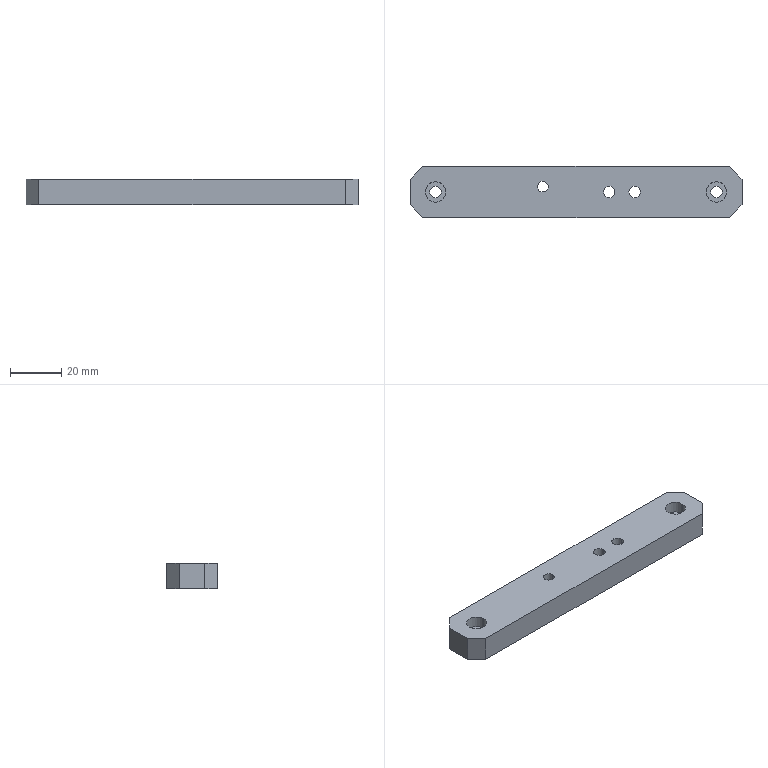Component | SolidWorks | P-SLJ-004-3_P-SLJ-004-003-1 | 1 solid | 32 faces | box 130 x 20 x 10 mm | volume 24093 mm3 | cylinder 18 | plane 14 | commonest cylinder face diameters 8 x8 4.5 x8 4.2 x2 | material A3
build123d program:
from build123d import *

# Parameters (mm, degrees)
SKETCH2_W                                            = 10
SKETCH2_H                                            = 20
EXTRUDE1_DEPTH                                       = 65
CBORE_FOR_M4_HEXAGON_SOCKET_HEAD_CAP_SCR_D           = 4.5
CBORE_FOR_M4_HEXAGON_SOCKET_HEAD_CAP_SCR_CBORE_D     = 8
CBORE_FOR_M4_HEXAGON_SOCKET_HEAD_CAP_SCR_CBORE_DEPTH = 4.6
M5_TAPPED_HOLE1_D                                    = 4.2
CBORE_FOR_M4_HEXAGON_SOCKET_HEAD_CAP_2_D             = 4.5
CBORE_FOR_M4_HEXAGON_SOCKET_HEAD_CAP_2_CBORE_D       = 8
CBORE_FOR_M4_HEXAGON_SOCKET_HEAD_CAP_2_CBORE_DEPTH   = 4.6
CHAMFER1_SIZE                                        = 5


with BuildPart() as part:
    # Sketch2 → Extrude1 (new, symmetric)
    with BuildSketch(Plane.XY):
        Rectangle(SKETCH2_W, SKETCH2_H)
    extrude(amount=EXTRUDE1_DEPTH, both=True)

    # CBORE for M4 Hexagon socket head cap scr (through all)
    with Locations(Plane.ZY.offset(5)):
        with Locations((-23, 0), (-13, 0)):
            CounterBoreHole(CBORE_FOR_M4_HEXAGON_SOCKET_HEAD_CAP_SCR_D / 2, CBORE_FOR_M4_HEXAGON_SOCKET_HEAD_CAP_SCR_CBORE_D / 2, CBORE_FOR_M4_HEXAGON_SOCKET_HEAD_CAP_SCR_CBORE_DEPTH)

    # M5 Tapped Hole1 (through all)
    with Locations(Plane.ZY.offset(5)):
        with Locations((13, 2.1)):
            Hole(M5_TAPPED_HOLE1_D / 2)

    # CBORE for M4 Hexagon socket head cap 2 (through all)
    with Locations(Plane(origin=(5, 2.408, 5.827), x_dir=(0, 0, 1), z_dir=(1, 0, 0))):
        with Locations((-60.827, 2.408), (49.173, 2.408)):
            CounterBoreHole(CBORE_FOR_M4_HEXAGON_SOCKET_HEAD_CAP_2_D / 2, CBORE_FOR_M4_HEXAGON_SOCKET_HEAD_CAP_2_CBORE_D / 2, CBORE_FOR_M4_HEXAGON_SOCKET_HEAD_CAP_2_CBORE_DEPTH)

    # Chamfer1
    chamfer1_edges = [part.edges().sort_by_distance(p)[0] for p in [
        (0, -10, 65),
        (0, -10, -65),
        (0, 10, -65),
        (0, 10, 65),
    ]]
    chamfer(chamfer1_edges, length=CHAMFER1_SIZE)


solid = part.part

# Placed as in the assembly
solid = solid.moved(Location((-219.5, -45, 1259.634), (0, -90, 0)))
STEP:
#1=CARTESIAN_POINT('',(-6.634,-1.772,49.608));
#2=VERTEX_POINT('',#1);
#3=CARTESIAN_POINT('',(-6.319,-1.772,49.608));
#4=VERTEX_POINT('',#3);
#5=CARTESIAN_POINT('',(-6.476,-1.772,49.608));
#6=DIRECTION('',(0.,-0.,1.));
#7=DIRECTION('',(1.,0.,0.));
#8=AXIS2_PLACEMENT_3D('',#5,#6,#7);
#9=CIRCLE('',#8,0.1575);
#10=EDGE_CURVE('',#2,#4,#9,.T.);
#11=ORIENTED_EDGE('',*,*,#10,.F.);
#12=CARTESIAN_POINT('',(-6.634,-1.772,49.789));
#13=VERTEX_POINT('',#12);
#14=CARTESIAN_POINT('',(-6.634,-1.772,49.789));
#15=DIRECTION('',(0.,-0.,1.));
#16=VECTOR('',#15,39.37);
#17=LINE('',#14,#16);
#18=EDGE_CURVE('',#2,#13,#17,.T.);
#19=ORIENTED_EDGE('',*,*,#18,.T.);
#20=CARTESIAN_POINT('',(-6.319,-1.772,49.789));
#21=VERTEX_POINT('',#20);
#22=CARTESIAN_POINT('',(-6.476,-1.772,49.789));
#23=DIRECTION('',(0.,-0.,1.));
#24=DIRECTION('',(1.,0.,0.));
#25=AXIS2_PLACEMENT_3D('',#22,#23,#24);
#26=CIRCLE('',#25,0.1575);
#27=EDGE_CURVE('',#13,#21,#26,.T.);
#28=ORIENTED_EDGE('',*,*,#27,.T.);
#29=CARTESIAN_POINT('',(-6.319,-1.772,49.789));
#30=DIRECTION('',(0.,-0.,1.));
#31=VECTOR('',#30,39.37);
#32=LINE('',#29,#31);
#33=EDGE_CURVE('',#4,#21,#32,.T.);
#34=ORIENTED_EDGE('',*,*,#33,.F.);
#35=EDGE_LOOP('',(#11,#19,#28,#34));
#36=FACE_OUTER_BOUND('',#35,.T.);
#37=CARTESIAN_POINT('',(-6.476,-1.772,49.789));
#38=DIRECTION('',(0.,-0.,1.));
#39=DIRECTION('',(1.,0.,0.));
#40=AXIS2_PLACEMENT_3D('',#37,#38,#39);
#41=CYLINDRICAL_SURFACE('',#40,0.1575);
#42=ADVANCED_FACE('',(#36),#41,.F.);
#43=CARTESIAN_POINT('',(-6.565,-1.772,49.395));
#44=VERTEX_POINT('',#43);
#45=CARTESIAN_POINT('',(-6.388,-1.772,49.395));
#46=VERTEX_POINT('',#45);
#47=CARTESIAN_POINT('',(-6.476,-1.772,49.395));
#48=DIRECTION('',(0.,-0.,1.));
#49=DIRECTION('',(1.,0.,0.));
#50=AXIS2_PLACEMENT_3D('',#47,#48,#49);
#51=CIRCLE('',#50,0.08858);
#52=EDGE_CURVE('',#44,#46,#51,.T.);
#53=ORIENTED_EDGE('',*,*,#52,.F.);
#54=CARTESIAN_POINT('',(-6.565,-1.772,49.608));
#55=VERTEX_POINT('',#54);
#56=CARTESIAN_POINT('',(-6.565,-1.772,49.789));
#57=DIRECTION('',(0.,-0.,1.));
#58=VECTOR('',#57,39.37);
#59=LINE('',#56,#58);
#60=EDGE_CURVE('',#44,#55,#59,.T.);
#61=ORIENTED_EDGE('',*,*,#60,.T.);
#62=CARTESIAN_POINT('',(-6.388,-1.772,49.608));
#63=VERTEX_POINT('',#62);
#64=CARTESIAN_POINT('',(-6.476,-1.772,49.608));
#65=DIRECTION('',(0.,-0.,1.));
#66=DIRECTION('',(1.,0.,0.));
#67=AXIS2_PLACEMENT_3D('',#64,#65,#66);
#68=CIRCLE('',#67,0.08858);
#69=EDGE_CURVE('',#55,#63,#68,.T.);
#70=ORIENTED_EDGE('',*,*,#69,.T.);
#71=CARTESIAN_POINT('',(-6.388,-1.772,49.789));
#72=DIRECTION('',(0.,-0.,1.));
#73=VECTOR('',#72,39.37);
#74=LINE('',#71,#73);
#75=EDGE_CURVE('',#46,#63,#74,.T.);
#76=ORIENTED_EDGE('',*,*,#75,.F.);
#77=EDGE_LOOP('',(#53,#61,#70,#76));
#78=FACE_OUTER_BOUND('',#77,.T.);
#79=CARTESIAN_POINT('',(-6.476,-1.772,49.789));
#80=DIRECTION('',(0.,-0.,1.));
#81=DIRECTION('',(1.,0.,0.));
#82=AXIS2_PLACEMENT_3D('',#79,#80,#81);
#83=CYLINDRICAL_SURFACE('',#82,0.08858);
#84=ADVANCED_FACE('',(#78),#83,.F.);
#85=CARTESIAN_POINT('',(-10.965,-1.772,49.608));
#86=VERTEX_POINT('',#85);
#87=CARTESIAN_POINT('',(-10.65,-1.772,49.608));
#88=VERTEX_POINT('',#87);
#89=CARTESIAN_POINT('',(-10.807,-1.772,49.608));
#90=DIRECTION('',(0.,-0.,1.));
#91=DIRECTION('',(1.,0.,0.));
#92=AXIS2_PLACEMENT_3D('',#89,#90,#91);
#93=CIRCLE('',#92,0.1575);
#94=EDGE_CURVE('',#86,#88,#93,.T.);
#95=ORIENTED_EDGE('',*,*,#94,.F.);
#96=CARTESIAN_POINT('',(-10.965,-1.772,49.789));
#97=VERTEX_POINT('',#96);
#98=CARTESIAN_POINT('',(-10.965,-1.772,49.789));
#99=DIRECTION('',(0.,-0.,1.));
#100=VECTOR('',#99,39.37);
#101=LINE('',#98,#100);
#102=EDGE_CURVE('',#86,#97,#101,.T.);
#103=ORIENTED_EDGE('',*,*,#102,.T.);
#104=CARTESIAN_POINT('',(-10.65,-1.772,49.789));
#105=VERTEX_POINT('',#104);
#106=CARTESIAN_POINT('',(-10.807,-1.772,49.789));
#107=DIRECTION('',(0.,-0.,1.));
#108=DIRECTION('',(1.,0.,0.));
#109=AXIS2_PLACEMENT_3D('',#106,#107,#108);
#110=CIRCLE('',#109,0.1575);
#111=EDGE_CURVE('',#97,#105,#110,.T.);
#112=ORIENTED_EDGE('',*,*,#111,.T.);
#113=CARTESIAN_POINT('',(-10.65,-1.772,49.789));
#114=DIRECTION('',(0.,-0.,1.));
#115=VECTOR('',#114,39.37);
#116=LINE('',#113,#115);
#117=EDGE_CURVE('',#88,#105,#116,.T.);
#118=ORIENTED_EDGE('',*,*,#117,.F.);
#119=EDGE_LOOP('',(#95,#103,#112,#118));
#120=FACE_OUTER_BOUND('',#119,.T.);
#121=CARTESIAN_POINT('',(-10.807,-1.772,49.789));
#122=DIRECTION('',(0.,-0.,1.));
#123=DIRECTION('',(1.,0.,0.));
#124=AXIS2_PLACEMENT_3D('',#121,#122,#123);
#125=CYLINDRICAL_SURFACE('',#124,0.1575);
#126=ADVANCED_FACE('',(#120),#125,.F.);
#127=CARTESIAN_POINT('',(-10.896,-1.772,49.395));
#128=VERTEX_POINT('',#127);
#129=CARTESIAN_POINT('',(-10.719,-1.772,49.395));
#130=VERTEX_POINT('',#129);
#131=CARTESIAN_POINT('',(-10.807,-1.772,49.395));
#132=DIRECTION('',(0.,-0.,1.));
#133=DIRECTION('',(1.,0.,0.));
#134=AXIS2_PLACEMENT_3D('',#131,#132,#133);
#135=CIRCLE('',#134,0.08858);
#136=EDGE_CURVE('',#128,#130,#135,.T.);
#137=ORIENTED_EDGE('',*,*,#136,.F.);
#138=CARTESIAN_POINT('',(-10.896,-1.772,49.608));
#139=VERTEX_POINT('',#138);
#140=CARTESIAN_POINT('',(-10.896,-1.772,49.789));
#141=DIRECTION('',(0.,-0.,1.));
#142=VECTOR('',#141,39.37);
#143=LINE('',#140,#142);
#144=EDGE_CURVE('',#128,#139,#143,.T.);
#145=ORIENTED_EDGE('',*,*,#144,.T.);
#146=CARTESIAN_POINT('',(-10.719,-1.772,49.608));
#147=VERTEX_POINT('',#146);
#148=CARTESIAN_POINT('',(-10.807,-1.772,49.608));
#149=DIRECTION('',(0.,-0.,1.));
#150=DIRECTION('',(1.,0.,0.));
#151=AXIS2_PLACEMENT_3D('',#148,#149,#150);
#152=CIRCLE('',#151,0.08858);
#153=EDGE_CURVE('',#139,#147,#152,.T.);
#154=ORIENTED_EDGE('',*,*,#153,.T.);
#155=CARTESIAN_POINT('',(-10.719,-1.772,49.789));
#156=DIRECTION('',(0.,-0.,1.));
#157=VECTOR('',#156,39.37);
#158=LINE('',#155,#157);
#159=EDGE_CURVE('',#130,#147,#158,.T.);
#160=ORIENTED_EDGE('',*,*,#159,.F.);
#161=EDGE_LOOP('',(#137,#145,#154,#160));
#162=FACE_OUTER_BOUND('',#161,.T.);
#163=CARTESIAN_POINT('',(-10.807,-1.772,49.789));
#164=DIRECTION('',(0.,-0.,1.));
#165=DIRECTION('',(1.,0.,0.));
#166=AXIS2_PLACEMENT_3D('',#163,#164,#165);
#167=CYLINDRICAL_SURFACE('',#166,0.08858);
#168=ADVANCED_FACE('',(#162),#167,.F.);
#169=CARTESIAN_POINT('',(-9.071,-1.689,49.789));
#170=VERTEX_POINT('',#169);
#171=CARTESIAN_POINT('',(-9.236,-1.689,49.789));
#172=VERTEX_POINT('',#171);
#173=CARTESIAN_POINT('',(-9.154,-1.689,49.789));
#174=DIRECTION('',(-0.,0.,-1.));
#175=DIRECTION('',(-1.,0.,0.));
#176=AXIS2_PLACEMENT_3D('',#173,#174,#175);
#177=CIRCLE('',#176,0.08268);
#178=EDGE_CURVE('',#170,#172,#177,.T.);
#179=ORIENTED_EDGE('',*,*,#178,.F.);
#180=CARTESIAN_POINT('',(-9.071,-1.689,49.395));
#181=VERTEX_POINT('',#180);
#182=CARTESIAN_POINT('',(-9.071,-1.689,49.395));
#183=DIRECTION('',(-0.,0.,-1.));
#184=VECTOR('',#183,39.37);
#185=LINE('',#182,#184);
#186=EDGE_CURVE('',#170,#181,#185,.T.);
#187=ORIENTED_EDGE('',*,*,#186,.T.);
#188=CARTESIAN_POINT('',(-9.236,-1.689,49.395));
#189=VERTEX_POINT('',#188);
#190=CARTESIAN_POINT('',(-9.154,-1.689,49.395));
#191=DIRECTION('',(-0.,0.,-1.));
#192=DIRECTION('',(-1.,0.,0.));
#193=AXIS2_PLACEMENT_3D('',#190,#191,#192);
#194=CIRCLE('',#193,0.08268);
#195=EDGE_CURVE('',#181,#189,#194,.T.);
#196=ORIENTED_EDGE('',*,*,#195,.T.);
#197=CARTESIAN_POINT('',(-9.236,-1.689,49.395));
#198=DIRECTION('',(-0.,0.,-1.));
#199=VECTOR('',#198,39.37);
#200=LINE('',#197,#199);
#201=EDGE_CURVE('',#172,#189,#200,.T.);
#202=ORIENTED_EDGE('',*,*,#201,.F.);
#203=EDGE_LOOP('',(#179,#187,#196,#202));
#204=FACE_OUTER_BOUND('',#203,.T.);
#205=CARTESIAN_POINT('',(-9.154,-1.689,49.395));
#206=DIRECTION('',(-0.,0.,-1.));
#207=DIRECTION('',(-1.,0.,0.));
#208=AXIS2_PLACEMENT_3D('',#205,#206,#207);
#209=CYLINDRICAL_SURFACE('',#208,0.08268);
#210=ADVANCED_FACE('',(#204),#209,.F.);
#211=CARTESIAN_POINT('',(-7.579,-1.772,49.576));
#212=VERTEX_POINT('',#211);
#213=CARTESIAN_POINT('',(-7.894,-1.772,49.576));
#214=VERTEX_POINT('',#213);
#215=CARTESIAN_POINT('',(-7.736,-1.772,49.576));
#216=DIRECTION('',(-0.,0.,-1.));
#217=DIRECTION('',(-1.,0.,0.));
#218=AXIS2_PLACEMENT_3D('',#215,#216,#217);
#219=CIRCLE('',#218,0.1575);
#220=EDGE_CURVE('',#212,#214,#219,.T.);
#221=ORIENTED_EDGE('',*,*,#220,.F.);
#222=CARTESIAN_POINT('',(-7.579,-1.772,49.395));
#223=VERTEX_POINT('',#222);
#224=CARTESIAN_POINT('',(-7.579,-1.772,49.395));
#225=DIRECTION('',(-0.,0.,-1.));
#226=VECTOR('',#225,39.37);
#227=LINE('',#224,#226);
#228=EDGE_CURVE('',#212,#223,#227,.T.);
#229=ORIENTED_EDGE('',*,*,#228,.T.);
#230=CARTESIAN_POINT('',(-7.894,-1.772,49.395));
#231=VERTEX_POINT('',#230);
#232=CARTESIAN_POINT('',(-7.736,-1.772,49.395));
#233=DIRECTION('',(-0.,0.,-1.));
#234=DIRECTION('',(-1.,0.,0.));
#235=AXIS2_PLACEMENT_3D('',#232,#233,#234);
#236=CIRCLE('',#235,0.1575);
#237=EDGE_CURVE('',#223,#231,#236,.T.);
#238=ORIENTED_EDGE('',*,*,#237,.T.);
#239=CARTESIAN_POINT('',(-7.894,-1.772,49.395));
#240=DIRECTION('',(-0.,0.,-1.));
#241=VECTOR('',#240,39.37);
#242=LINE('',#239,#241);
#243=EDGE_CURVE('',#214,#231,#242,.T.);
#244=ORIENTED_EDGE('',*,*,#243,.F.);
#245=EDGE_LOOP('',(#221,#229,#238,#244));
#246=FACE_OUTER_BOUND('',#245,.T.);
#247=CARTESIAN_POINT('',(-7.736,-1.772,49.395));
#248=DIRECTION('',(-0.,0.,-1.));
#249=DIRECTION('',(-1.,0.,0.));
#250=AXIS2_PLACEMENT_3D('',#247,#248,#249);
#251=CYLINDRICAL_SURFACE('',#250,0.1575);
#252=ADVANCED_FACE('',(#246),#251,.F.);
#253=CARTESIAN_POINT('',(-7.648,-1.772,49.789));
#254=VERTEX_POINT('',#253);
#255=CARTESIAN_POINT('',(-7.825,-1.772,49.789));
#256=VERTEX_POINT('',#255);
#257=CARTESIAN_POINT('',(-7.736,-1.772,49.789));
#258=DIRECTION('',(-0.,0.,-1.));
#259=DIRECTION('',(-1.,0.,0.));
#260=AXIS2_PLACEMENT_3D('',#257,#258,#259);
#261=CIRCLE('',#260,0.08858);
#262=EDGE_CURVE('',#254,#256,#261,.T.);
#263=ORIENTED_EDGE('',*,*,#262,.F.);
#264=CARTESIAN_POINT('',(-7.648,-1.772,49.576));
#265=VERTEX_POINT('',#264);
#266=CARTESIAN_POINT('',(-7.648,-1.772,49.395));
#267=DIRECTION('',(-0.,0.,-1.));
#268=VECTOR('',#267,39.37);
#269=LINE('',#266,#268);
#270=EDGE_CURVE('',#254,#265,#269,.T.);
#271=ORIENTED_EDGE('',*,*,#270,.T.);
#272=CARTESIAN_POINT('',(-7.825,-1.772,49.576));
#273=VERTEX_POINT('',#272);
#274=CARTESIAN_POINT('',(-7.736,-1.772,49.576));
#275=DIRECTION('',(-0.,0.,-1.));
#276=DIRECTION('',(-1.,0.,0.));
#277=AXIS2_PLACEMENT_3D('',#274,#275,#276);
#278=CIRCLE('',#277,0.08858);
#279=EDGE_CURVE('',#265,#273,#278,.T.);
#280=ORIENTED_EDGE('',*,*,#279,.T.);
#281=CARTESIAN_POINT('',(-7.825,-1.772,49.395));
#282=DIRECTION('',(-0.,0.,-1.));
#283=VECTOR('',#282,39.37);
#284=LINE('',#281,#283);
#285=EDGE_CURVE('',#256,#273,#284,.T.);
#286=ORIENTED_EDGE('',*,*,#285,.F.);
#287=EDGE_LOOP('',(#263,#271,#280,#286));
#288=FACE_OUTER_BOUND('',#287,.T.);
#289=CARTESIAN_POINT('',(-7.736,-1.772,49.395));
#290=DIRECTION('',(-0.,0.,-1.));
#291=DIRECTION('',(-1.,0.,0.));
#292=AXIS2_PLACEMENT_3D('',#289,#290,#291);
#293=CYLINDRICAL_SURFACE('',#292,0.08858);
#294=ADVANCED_FACE('',(#288),#293,.F.);
#295=CARTESIAN_POINT('',(-7.972,-1.772,49.576));
#296=VERTEX_POINT('',#295);
#297=CARTESIAN_POINT('',(-8.287,-1.772,49.576));
#298=VERTEX_POINT('',#297);
#299=CARTESIAN_POINT('',(-8.13,-1.772,49.576));
#300=DIRECTION('',(-0.,0.,-1.));
#301=DIRECTION('',(-1.,0.,0.));
#302=AXIS2_PLACEMENT_3D('',#299,#300,#301);
#303=CIRCLE('',#302,0.1575);
#304=EDGE_CURVE('',#296,#298,#303,.T.);
#305=ORIENTED_EDGE('',*,*,#304,.F.);
#306=CARTESIAN_POINT('',(-7.972,-1.772,49.395));
#307=VERTEX_POINT('',#306);
#308=CARTESIAN_POINT('',(-7.972,-1.772,49.395));
#309=DIRECTION('',(-0.,0.,-1.));
#310=VECTOR('',#309,39.37);
#311=LINE('',#308,#310);
#312=EDGE_CURVE('',#296,#307,#311,.T.);
#313=ORIENTED_EDGE('',*,*,#312,.T.);
#314=CARTESIAN_POINT('',(-8.287,-1.772,49.395));
#315=VERTEX_POINT('',#314);
#316=CARTESIAN_POINT('',(-8.13,-1.772,49.395));
#317=DIRECTION('',(-0.,0.,-1.));
#318=DIRECTION('',(-1.,0.,0.));
#319=AXIS2_PLACEMENT_3D('',#316,#317,#318);
#320=CIRCLE('',#319,0.1575);
#321=EDGE_CURVE('',#307,#315,#320,.T.);
#322=ORIENTED_EDGE('',*,*,#321,.T.);
#323=CARTESIAN_POINT('',(-8.287,-1.772,49.395));
#324=DIRECTION('',(-0.,0.,-1.));
#325=VECTOR('',#324,39.37);
#326=LINE('',#323,#325);
#327=EDGE_CURVE('',#298,#315,#326,.T.);
#328=ORIENTED_EDGE('',*,*,#327,.F.);
#329=EDGE_LOOP('',(#305,#313,#322,#328));
#330=FACE_OUTER_BOUND('',#329,.T.);
#331=CARTESIAN_POINT('',(-8.13,-1.772,49.395));
#332=DIRECTION('',(-0.,0.,-1.));
#333=DIRECTION('',(-1.,0.,0.));
#334=AXIS2_PLACEMENT_3D('',#331,#332,#333);
#335=CYLINDRICAL_SURFACE('',#334,0.1575);
#336=ADVANCED_FACE('',(#330),#335,.F.);
#337=CARTESIAN_POINT('',(-8.041,-1.772,49.789));
#338=VERTEX_POINT('',#337);
#339=CARTESIAN_POINT('',(-8.219,-1.772,49.789));
#340=VERTEX_POINT('',#339);
#341=CARTESIAN_POINT('',(-8.13,-1.772,49.789));
#342=DIRECTION('',(-0.,0.,-1.));
#343=DIRECTION('',(-1.,0.,0.));
#344=AXIS2_PLACEMENT_3D('',#341,#342,#343);
#345=CIRCLE('',#344,0.08858);
#346=EDGE_CURVE('',#338,#340,#345,.T.);
#347=ORIENTED_EDGE('',*,*,#346,.F.);
#348=CARTESIAN_POINT('',(-8.041,-1.772,49.576));
#349=VERTEX_POINT('',#348);
#350=CARTESIAN_POINT('',(-8.041,-1.772,49.395));
#351=DIRECTION('',(-0.,0.,-1.));
#352=VECTOR('',#351,39.37);
#353=LINE('',#350,#352);
#354=EDGE_CURVE('',#338,#349,#353,.T.);
#355=ORIENTED_EDGE('',*,*,#354,.T.);
#356=CARTESIAN_POINT('',(-8.219,-1.772,49.576));
#357=VERTEX_POINT('',#356);
#358=CARTESIAN_POINT('',(-8.13,-1.772,49.576));
#359=DIRECTION('',(-0.,0.,-1.));
#360=DIRECTION('',(-1.,0.,0.));
#361=AXIS2_PLACEMENT_3D('',#358,#359,#360);
#362=CIRCLE('',#361,0.08858);
#363=EDGE_CURVE('',#349,#357,#362,.T.);
#364=ORIENTED_EDGE('',*,*,#363,.T.);
#365=CARTESIAN_POINT('',(-8.219,-1.772,49.395));
#366=DIRECTION('',(-0.,0.,-1.));
#367=VECTOR('',#366,39.37);
#368=LINE('',#365,#367);
#369=EDGE_CURVE('',#340,#357,#368,.T.);
#370=ORIENTED_EDGE('',*,*,#369,.F.);
#371=EDGE_LOOP('',(#347,#355,#364,#370));
#372=FACE_OUTER_BOUND('',#371,.T.);
#373=CARTESIAN_POINT('',(-8.13,-1.772,49.395));
#374=DIRECTION('',(-0.,0.,-1.));
#375=DIRECTION('',(-1.,0.,0.));
#376=AXIS2_PLACEMENT_3D('',#373,#374,#375);
#377=CYLINDRICAL_SURFACE('',#376,0.08858);
#378=ADVANCED_FACE('',(#372),#377,.F.);
#379=CARTESIAN_POINT('',(-6.476,-1.772,49.789));
#380=DIRECTION('',(0.,-0.,1.));
#381=DIRECTION('',(1.,0.,0.));
#382=AXIS2_PLACEMENT_3D('',#379,#380,#381);
#383=CIRCLE('',#382,0.1575);
#384=EDGE_CURVE('',#21,#13,#383,.T.);
#385=ORIENTED_EDGE('',*,*,#384,.F.);
#386=ORIENTED_EDGE('',*,*,#27,.F.);
#387=EDGE_LOOP('',(#385,#386));
#388=FACE_BOUND('',#387,.T.);
#389=CARTESIAN_POINT('',(-10.807,-1.772,49.789));
#390=DIRECTION('',(0.,-0.,1.));
#391=DIRECTION('',(1.,0.,0.));
#392=AXIS2_PLACEMENT_3D('',#389,#390,#391);
#393=CIRCLE('',#392,0.1575);
#394=EDGE_CURVE('',#105,#97,#393,.T.);
#395=ORIENTED_EDGE('',*,*,#394,.F.);
#396=ORIENTED_EDGE('',*,*,#111,.F.);
#397=EDGE_LOOP('',(#395,#396));
#398=FACE_BOUND('',#397,.T.);
#399=CARTESIAN_POINT('',(-9.154,-1.689,49.789));
#400=DIRECTION('',(-0.,0.,-1.));
#401=DIRECTION('',(-1.,0.,0.));
#402=AXIS2_PLACEMENT_3D('',#399,#400,#401);
#403=CIRCLE('',#402,0.08268);
#404=EDGE_CURVE('',#172,#170,#403,.T.);
#405=ORIENTED_EDGE('',*,*,#404,.T.);
#406=ORIENTED_EDGE('',*,*,#178,.T.);
#407=EDGE_LOOP('',(#405,#406));
#408=FACE_BOUND('',#407,.T.);
#409=CARTESIAN_POINT('',(-7.736,-1.772,49.789));
#410=DIRECTION('',(-0.,0.,-1.));
#411=DIRECTION('',(-1.,0.,0.));
#412=AXIS2_PLACEMENT_3D('',#409,#410,#411);
#413=CIRCLE('',#412,0.08858);
#414=EDGE_CURVE('',#256,#254,#413,.T.);
#415=ORIENTED_EDGE('',*,*,#414,.T.);
#416=ORIENTED_EDGE('',*,*,#262,.T.);
#417=EDGE_LOOP('',(#415,#416));
#418=FACE_BOUND('',#417,.T.);
#419=CARTESIAN_POINT('',(-8.13,-1.772,49.789));
#420=DIRECTION('',(-0.,0.,-1.));
#421=DIRECTION('',(-1.,0.,0.));
#422=AXIS2_PLACEMENT_3D('',#419,#420,#421);
#423=CIRCLE('',#422,0.08858);
#424=EDGE_CURVE('',#340,#338,#423,.T.);
#425=ORIENTED_EDGE('',*,*,#424,.T.);
#426=ORIENTED_EDGE('',*,*,#346,.T.);
#427=EDGE_LOOP('',(#425,#426));
#428=FACE_BOUND('',#427,.T.);
#429=CARTESIAN_POINT('',(-11.201,-1.969,49.789));
#430=VERTEX_POINT('',#429);
#431=CARTESIAN_POINT('',(-11.201,-1.575,49.789));
#432=VERTEX_POINT('',#431);
#433=CARTESIAN_POINT('',(-11.201,-2.165,49.789));
#434=DIRECTION('',(0.,1.,0.));
#435=VECTOR('',#434,39.37);
#436=LINE('',#433,#435);
#437=EDGE_CURVE('',#430,#432,#436,.T.);
#438=ORIENTED_EDGE('',*,*,#437,.F.);
#439=CARTESIAN_POINT('',(-11.004,-2.165,49.789));
#440=VERTEX_POINT('',#439);
#441=CARTESIAN_POINT('',(-11.201,-1.969,49.789));
#442=DIRECTION('',(0.7071,-0.7071,-0.));
#443=VECTOR('',#442,39.37);
#444=LINE('',#441,#443);
#445=EDGE_CURVE('',#430,#440,#444,.T.);
#446=ORIENTED_EDGE('',*,*,#445,.T.);
#447=CARTESIAN_POINT('',(-6.28,-2.165,49.789));
#448=VERTEX_POINT('',#447);
#449=CARTESIAN_POINT('',(-11.201,-2.165,49.789));
#450=DIRECTION('',(1.,-0.,-0.));
#451=VECTOR('',#450,39.37);
#452=LINE('',#449,#451);
#453=EDGE_CURVE('',#440,#448,#452,.T.);
#454=ORIENTED_EDGE('',*,*,#453,.T.);
#455=CARTESIAN_POINT('',(-6.083,-1.969,49.789));
#456=VERTEX_POINT('',#455);
#457=CARTESIAN_POINT('',(-6.28,-2.165,49.789));
#458=DIRECTION('',(0.7071,0.7071,0.));
#459=VECTOR('',#458,39.37);
#460=LINE('',#457,#459);
#461=EDGE_CURVE('',#448,#456,#460,.T.);
#462=ORIENTED_EDGE('',*,*,#461,.T.);
#463=CARTESIAN_POINT('',(-6.083,-1.575,49.789));
#464=VERTEX_POINT('',#463);
#465=CARTESIAN_POINT('',(-6.083,-2.165,49.789));
#466=DIRECTION('',(0.,1.,0.));
#467=VECTOR('',#466,39.37);
#468=LINE('',#465,#467);
#469=EDGE_CURVE('',#456,#464,#468,.T.);
#470=ORIENTED_EDGE('',*,*,#469,.T.);
#471=CARTESIAN_POINT('',(-6.28,-1.378,49.789));
#472=VERTEX_POINT('',#471);
#473=CARTESIAN_POINT('',(-6.28,-1.378,49.789));
#474=DIRECTION('',(-0.7071,0.7071,0.));
#475=VECTOR('',#474,39.37);
#476=LINE('',#473,#475);
#477=EDGE_CURVE('',#464,#472,#476,.T.);
#478=ORIENTED_EDGE('',*,*,#477,.T.);
#479=CARTESIAN_POINT('',(-11.004,-1.378,49.789));
#480=VERTEX_POINT('',#479);
#481=CARTESIAN_POINT('',(-11.201,-1.378,49.789));
#482=DIRECTION('',(1.,-0.,-0.));
#483=VECTOR('',#482,39.37);
#484=LINE('',#481,#483);
#485=EDGE_CURVE('',#480,#472,#484,.T.);
#486=ORIENTED_EDGE('',*,*,#485,.F.);
#487=CARTESIAN_POINT('',(-11.201,-1.575,49.789));
#488=DIRECTION('',(-0.7071,-0.7071,-0.));
#489=VECTOR('',#488,39.37);
#490=LINE('',#487,#489);
#491=EDGE_CURVE('',#480,#432,#490,.T.);
#492=ORIENTED_EDGE('',*,*,#491,.T.);
#493=EDGE_LOOP('',(#438,#446,#454,#462,#470,#478,#486,#492));
#494=FACE_OUTER_BOUND('',#493,.T.);
#495=CARTESIAN_POINT('',(-11.201,-2.165,49.789));
#496=DIRECTION('',(-0.,0.,-1.));
#497=DIRECTION('',(-1.,0.,0.));
#498=AXIS2_PLACEMENT_3D('',#495,#496,#497);
#499=PLANE('',#498);
#500=ADVANCED_FACE('',(#388,#398,#408,#418,#428,#494),#499,.F.);
#501=CARTESIAN_POINT('',(-11.004,-1.378,49.395));
#502=VERTEX_POINT('',#501);
#503=CARTESIAN_POINT('',(-6.28,-1.378,49.395));
#504=VERTEX_POINT('',#503);
#505=CARTESIAN_POINT('',(-11.201,-1.378,49.395));
#506=DIRECTION('',(1.,-0.,-0.));
#507=VECTOR('',#506,39.37);
#508=LINE('',#505,#507);
#509=EDGE_CURVE('',#502,#504,#508,.T.);
#510=ORIENTED_EDGE('',*,*,#509,.F.);
#511=CARTESIAN_POINT('',(-11.004,-1.378,49.395));
#512=DIRECTION('',(0.,-0.,1.));
#513=VECTOR('',#512,39.37);
#514=LINE('',#511,#513);
#515=EDGE_CURVE('',#502,#480,#514,.T.);
#516=ORIENTED_EDGE('',*,*,#515,.T.);
#517=ORIENTED_EDGE('',*,*,#485,.T.);
#518=CARTESIAN_POINT('',(-6.28,-1.378,49.395));
#519=DIRECTION('',(-0.,0.,-1.));
#520=VECTOR('',#519,39.37);
#521=LINE('',#518,#520);
#522=EDGE_CURVE('',#472,#504,#521,.T.);
#523=ORIENTED_EDGE('',*,*,#522,.T.);
#524=EDGE_LOOP('',(#510,#516,#517,#523));
#525=FACE_OUTER_BOUND('',#524,.T.);
#526=CARTESIAN_POINT('',(-11.201,-1.378,49.395));
#527=DIRECTION('',(-0.,-1.,-0.));
#528=DIRECTION('',(1.,-0.,-0.));
#529=AXIS2_PLACEMENT_3D('',#526,#527,#528);
#530=PLANE('',#529);
#531=ADVANCED_FACE('',(#525),#530,.F.);
#532=CARTESIAN_POINT('',(-6.476,-1.772,49.395));
#533=DIRECTION('',(0.,-0.,1.));
#534=DIRECTION('',(1.,0.,0.));
#535=AXIS2_PLACEMENT_3D('',#532,#533,#534);
#536=CIRCLE('',#535,0.08858);
#537=EDGE_CURVE('',#46,#44,#536,.T.);
#538=ORIENTED_EDGE('',*,*,#537,.T.);
#539=ORIENTED_EDGE('',*,*,#52,.T.);
#540=EDGE_LOOP('',(#538,#539));
#541=FACE_BOUND('',#540,.T.);
#542=CARTESIAN_POINT('',(-10.807,-1.772,49.395));
#543=DIRECTION('',(0.,-0.,1.));
#544=DIRECTION('',(1.,0.,0.));
#545=AXIS2_PLACEMENT_3D('',#542,#543,#544);
#546=CIRCLE('',#545,0.08858);
#547=EDGE_CURVE('',#130,#128,#546,.T.);
#548=ORIENTED_EDGE('',*,*,#547,.T.);
#549=ORIENTED_EDGE('',*,*,#136,.T.);
#550=EDGE_LOOP('',(#548,#549));
#551=FACE_BOUND('',#550,.T.);
#552=CARTESIAN_POINT('',(-9.154,-1.689,49.395));
#553=DIRECTION('',(-0.,0.,-1.));
#554=DIRECTION('',(-1.,0.,0.));
#555=AXIS2_PLACEMENT_3D('',#552,#553,#554);
#556=CIRCLE('',#555,0.08268);
#557=EDGE_CURVE('',#189,#181,#556,.T.);
#558=ORIENTED_EDGE('',*,*,#557,.F.);
#559=ORIENTED_EDGE('',*,*,#195,.F.);
#560=EDGE_LOOP('',(#558,#559));
#561=FACE_BOUND('',#560,.T.);
#562=CARTESIAN_POINT('',(-7.736,-1.772,49.395));
#563=DIRECTION('',(-0.,0.,-1.));
#564=DIRECTION('',(-1.,0.,0.));
#565=AXIS2_PLACEMENT_3D('',#562,#563,#564);
#566=CIRCLE('',#565,0.1575);
#567=EDGE_CURVE('',#231,#223,#566,.T.);
#568=ORIENTED_EDGE('',*,*,#567,.F.);
#569=ORIENTED_EDGE('',*,*,#237,.F.);
#570=EDGE_LOOP('',(#568,#569));
#571=FACE_BOUND('',#570,.T.);
#572=CARTESIAN_POINT('',(-8.13,-1.772,49.395));
#573=DIRECTION('',(-0.,0.,-1.));
#574=DIRECTION('',(-1.,0.,0.));
#575=AXIS2_PLACEMENT_3D('',#572,#573,#574);
#576=CIRCLE('',#575,0.1575);
#577=EDGE_CURVE('',#315,#307,#576,.T.);
#578=ORIENTED_EDGE('',*,*,#577,.F.);
#579=ORIENTED_EDGE('',*,*,#321,.F.);
#580=EDGE_LOOP('',(#578,#579));
#581=FACE_BOUND('',#580,.T.);
#582=CARTESIAN_POINT('',(-11.004,-2.165,49.395));
#583=VERTEX_POINT('',#582);
#584=CARTESIAN_POINT('',(-6.28,-2.165,49.395));
#585=VERTEX_POINT('',#584);
#586=CARTESIAN_POINT('',(-11.201,-2.165,49.395));
#587=DIRECTION('',(1.,-0.,-0.));
#588=VECTOR('',#587,39.37);
#589=LINE('',#586,#588);
#590=EDGE_CURVE('',#583,#585,#589,.T.);
#591=ORIENTED_EDGE('',*,*,#590,.F.);
#592=CARTESIAN_POINT('',(-11.201,-1.969,49.395));
#593=VERTEX_POINT('',#592);
#594=CARTESIAN_POINT('',(-11.201,-1.969,49.395));
#595=DIRECTION('',(-0.7071,0.7071,0.));
#596=VECTOR('',#595,39.37);
#597=LINE('',#594,#596);
#598=EDGE_CURVE('',#583,#593,#597,.T.);
#599=ORIENTED_EDGE('',*,*,#598,.T.);
#600=CARTESIAN_POINT('',(-11.201,-1.575,49.395));
#601=VERTEX_POINT('',#600);
#602=CARTESIAN_POINT('',(-11.201,-2.165,49.395));
#603=DIRECTION('',(-0.,-1.,-0.));
#604=VECTOR('',#603,39.37);
#605=LINE('',#602,#604);
#606=EDGE_CURVE('',#601,#593,#605,.T.);
#607=ORIENTED_EDGE('',*,*,#606,.F.);
#608=CARTESIAN_POINT('',(-11.201,-1.575,49.395));
#609=DIRECTION('',(0.7071,0.7071,0.));
#610=VECTOR('',#609,39.37);
#611=LINE('',#608,#610);
#612=EDGE_CURVE('',#601,#502,#611,.T.);
#613=ORIENTED_EDGE('',*,*,#612,.T.);
#614=ORIENTED_EDGE('',*,*,#509,.T.);
#615=CARTESIAN_POINT('',(-6.083,-1.575,49.395));
#616=VERTEX_POINT('',#615);
#617=CARTESIAN_POINT('',(-6.28,-1.378,49.395));
#618=DIRECTION('',(0.7071,-0.7071,-0.));
#619=VECTOR('',#618,39.37);
#620=LINE('',#617,#619);
#621=EDGE_CURVE('',#504,#616,#620,.T.);
#622=ORIENTED_EDGE('',*,*,#621,.T.);
#623=CARTESIAN_POINT('',(-6.083,-1.969,49.395));
#624=VERTEX_POINT('',#623);
#625=CARTESIAN_POINT('',(-6.083,-2.165,49.395));
#626=DIRECTION('',(-0.,-1.,-0.));
#627=VECTOR('',#626,39.37);
#628=LINE('',#625,#627);
#629=EDGE_CURVE('',#616,#624,#628,.T.);
#630=ORIENTED_EDGE('',*,*,#629,.T.);
#631=CARTESIAN_POINT('',(-6.28,-2.165,49.395));
#632=DIRECTION('',(-0.7071,-0.7071,-0.));
#633=VECTOR('',#632,39.37);
#634=LINE('',#631,#633);
#635=EDGE_CURVE('',#624,#585,#634,.T.);
#636=ORIENTED_EDGE('',*,*,#635,.T.);
#637=EDGE_LOOP('',(#591,#599,#607,#613,#614,#622,#630,#636));
#638=FACE_OUTER_BOUND('',#637,.T.);
#639=CARTESIAN_POINT('',(-11.201,-2.165,49.395));
#640=DIRECTION('',(0.,-0.,1.));
#641=DIRECTION('',(1.,-0.,-0.));
#642=AXIS2_PLACEMENT_3D('',#639,#640,#641);
#643=PLANE('',#642);
#644=ADVANCED_FACE('',(#541,#551,#561,#571,#581,#638),#643,.F.);
#645=ORIENTED_EDGE('',*,*,#453,.F.);
#646=CARTESIAN_POINT('',(-11.004,-2.165,49.395));
#647=DIRECTION('',(-0.,0.,-1.));
#648=VECTOR('',#647,39.37);
#649=LINE('',#646,#648);
#650=EDGE_CURVE('',#440,#583,#649,.T.);
#651=ORIENTED_EDGE('',*,*,#650,.T.);
#652=ORIENTED_EDGE('',*,*,#590,.T.);
#653=CARTESIAN_POINT('',(-6.28,-2.165,49.789));
#654=DIRECTION('',(0.,-0.,1.));
#655=VECTOR('',#654,39.37);
#656=LINE('',#653,#655);
#657=EDGE_CURVE('',#585,#448,#656,.T.);
#658=ORIENTED_EDGE('',*,*,#657,.T.);
#659=EDGE_LOOP('',(#645,#651,#652,#658));
#660=FACE_OUTER_BOUND('',#659,.T.);
#661=CARTESIAN_POINT('',(-11.201,-2.165,49.395));
#662=DIRECTION('',(0.,1.,0.));
#663=DIRECTION('',(-1.,0.,0.));
#664=AXIS2_PLACEMENT_3D('',#661,#662,#663);
#665=PLANE('',#664);
#666=ADVANCED_FACE('',(#660),#665,.F.);
#667=ORIENTED_EDGE('',*,*,#606,.T.);
#668=CARTESIAN_POINT('',(-11.201,-1.969,49.592));
#669=DIRECTION('',(0.,-0.,1.));
#670=VECTOR('',#669,39.37);
#671=LINE('',#668,#670);
#672=EDGE_CURVE('',#593,#430,#671,.T.);
#673=ORIENTED_EDGE('',*,*,#672,.T.);
#674=ORIENTED_EDGE('',*,*,#437,.T.);
#675=CARTESIAN_POINT('',(-11.201,-1.575,49.592));
#676=DIRECTION('',(-0.,0.,-1.));
#677=VECTOR('',#676,39.37);
#678=LINE('',#675,#677);
#679=EDGE_CURVE('',#432,#601,#678,.T.);
#680=ORIENTED_EDGE('',*,*,#679,.T.);
#681=EDGE_LOOP('',(#667,#673,#674,#680));
#682=FACE_OUTER_BOUND('',#681,.T.);
#683=CARTESIAN_POINT('',(-11.201,-1.772,49.592));
#684=DIRECTION('',(1.,-0.,-0.));
#685=DIRECTION('',(-0.,0.,-1.));
#686=AXIS2_PLACEMENT_3D('',#683,#684,#685);
#687=PLANE('',#686);
#688=ADVANCED_FACE('',(#682),#687,.F.);
#689=ORIENTED_EDGE('',*,*,#469,.F.);
#690=CARTESIAN_POINT('',(-6.083,-1.969,49.395));
#691=DIRECTION('',(-0.,0.,-1.));
#692=VECTOR('',#691,39.37);
#693=LINE('',#690,#692);
#694=EDGE_CURVE('',#456,#624,#693,.T.);
#695=ORIENTED_EDGE('',*,*,#694,.T.);
#696=ORIENTED_EDGE('',*,*,#629,.F.);
#697=CARTESIAN_POINT('',(-6.083,-1.575,49.789));
#698=DIRECTION('',(0.,-0.,1.));
#699=VECTOR('',#698,39.37);
#700=LINE('',#697,#699);
#701=EDGE_CURVE('',#616,#464,#700,.T.);
#702=ORIENTED_EDGE('',*,*,#701,.T.);
#703=EDGE_LOOP('',(#689,#695,#696,#702));
#704=FACE_OUTER_BOUND('',#703,.T.);
#705=CARTESIAN_POINT('',(-6.083,-1.772,49.592));
#706=DIRECTION('',(1.,-0.,-0.));
#707=DIRECTION('',(-0.,0.,-1.));
#708=AXIS2_PLACEMENT_3D('',#705,#706,#707);
#709=PLANE('',#708);
#710=ADVANCED_FACE('',(#704),#709,.T.);
#711=ORIENTED_EDGE('',*,*,#354,.F.);
#712=ORIENTED_EDGE('',*,*,#424,.F.);
#713=ORIENTED_EDGE('',*,*,#369,.T.);
#714=CARTESIAN_POINT('',(-8.13,-1.772,49.576));
#715=DIRECTION('',(-0.,0.,-1.));
#716=DIRECTION('',(-1.,0.,0.));
#717=AXIS2_PLACEMENT_3D('',#714,#715,#716);
#718=CIRCLE('',#717,0.08858);
#719=EDGE_CURVE('',#357,#349,#718,.T.);
#720=ORIENTED_EDGE('',*,*,#719,.T.);
#721=EDGE_LOOP('',(#711,#712,#713,#720));
#722=FACE_OUTER_BOUND('',#721,.T.);
#723=CARTESIAN_POINT('',(-8.13,-1.772,49.395));
#724=DIRECTION('',(-0.,0.,-1.));
#725=DIRECTION('',(-1.,0.,0.));
#726=AXIS2_PLACEMENT_3D('',#723,#724,#725);
#727=CYLINDRICAL_SURFACE('',#726,0.08858);
#728=ADVANCED_FACE('',(#722),#727,.F.);
#729=ORIENTED_EDGE('',*,*,#719,.F.);
#730=ORIENTED_EDGE('',*,*,#363,.F.);
#731=EDGE_LOOP('',(#729,#730));
#732=FACE_BOUND('',#731,.T.);
#733=CARTESIAN_POINT('',(-8.13,-1.772,49.576));
#734=DIRECTION('',(-0.,0.,-1.));
#735=DIRECTION('',(-1.,0.,0.));
#736=AXIS2_PLACEMENT_3D('',#733,#734,#735);
#737=CIRCLE('',#736,0.1575);
#738=EDGE_CURVE('',#298,#296,#737,.T.);
#739=ORIENTED_EDGE('',*,*,#738,.T.);
#740=ORIENTED_EDGE('',*,*,#304,.T.);
#741=EDGE_LOOP('',(#739,#740));
#742=FACE_OUTER_BOUND('',#741,.T.);
#743=CARTESIAN_POINT('',(-8.13,-1.683,49.576));
#744=DIRECTION('',(0.,-0.,1.));
#745=DIRECTION('',(1.,-0.,-0.));
#746=AXIS2_PLACEMENT_3D('',#743,#744,#745);
#747=PLANE('',#746);
#748=ADVANCED_FACE('',(#732,#742),#747,.F.);
#749=ORIENTED_EDGE('',*,*,#312,.F.);
#750=ORIENTED_EDGE('',*,*,#738,.F.);
#751=ORIENTED_EDGE('',*,*,#327,.T.);
#752=ORIENTED_EDGE('',*,*,#577,.T.);
#753=EDGE_LOOP('',(#749,#750,#751,#752));
#754=FACE_OUTER_BOUND('',#753,.T.);
#755=CARTESIAN_POINT('',(-8.13,-1.772,49.395));
#756=DIRECTION('',(-0.,0.,-1.));
#757=DIRECTION('',(-1.,0.,0.));
#758=AXIS2_PLACEMENT_3D('',#755,#756,#757);
#759=CYLINDRICAL_SURFACE('',#758,0.1575);
#760=ADVANCED_FACE('',(#754),#759,.F.);
#761=ORIENTED_EDGE('',*,*,#270,.F.);
#762=ORIENTED_EDGE('',*,*,#414,.F.);
#763=ORIENTED_EDGE('',*,*,#285,.T.);
#764=CARTESIAN_POINT('',(-7.736,-1.772,49.576));
#765=DIRECTION('',(-0.,0.,-1.));
#766=DIRECTION('',(-1.,0.,0.));
#767=AXIS2_PLACEMENT_3D('',#764,#765,#766);
#768=CIRCLE('',#767,0.08858);
#769=EDGE_CURVE('',#273,#265,#768,.T.);
#770=ORIENTED_EDGE('',*,*,#769,.T.);
#771=EDGE_LOOP('',(#761,#762,#763,#770));
#772=FACE_OUTER_BOUND('',#771,.T.);
#773=CARTESIAN_POINT('',(-7.736,-1.772,49.395));
#774=DIRECTION('',(-0.,0.,-1.));
#775=DIRECTION('',(-1.,0.,0.));
#776=AXIS2_PLACEMENT_3D('',#773,#774,#775);
#777=CYLINDRICAL_SURFACE('',#776,0.08858);
#778=ADVANCED_FACE('',(#772),#777,.F.);
#779=ORIENTED_EDGE('',*,*,#769,.F.);
#780=ORIENTED_EDGE('',*,*,#279,.F.);
#781=EDGE_LOOP('',(#779,#780));
#782=FACE_BOUND('',#781,.T.);
#783=CARTESIAN_POINT('',(-7.736,-1.772,49.576));
#784=DIRECTION('',(-0.,0.,-1.));
#785=DIRECTION('',(-1.,0.,0.));
#786=AXIS2_PLACEMENT_3D('',#783,#784,#785);
#787=CIRCLE('',#786,0.1575);
#788=EDGE_CURVE('',#214,#212,#787,.T.);
#789=ORIENTED_EDGE('',*,*,#788,.T.);
#790=ORIENTED_EDGE('',*,*,#220,.T.);
#791=EDGE_LOOP('',(#789,#790));
#792=FACE_OUTER_BOUND('',#791,.T.);
#793=CARTESIAN_POINT('',(-7.736,-1.683,49.576));
#794=DIRECTION('',(0.,-0.,1.));
#795=DIRECTION('',(1.,-0.,-0.));
#796=AXIS2_PLACEMENT_3D('',#793,#794,#795);
#797=PLANE('',#796);
#798=ADVANCED_FACE('',(#782,#792),#797,.F.);
#799=ORIENTED_EDGE('',*,*,#228,.F.);
#800=ORIENTED_EDGE('',*,*,#788,.F.);
#801=ORIENTED_EDGE('',*,*,#243,.T.);
#802=ORIENTED_EDGE('',*,*,#567,.T.);
#803=EDGE_LOOP('',(#799,#800,#801,#802));
#804=FACE_OUTER_BOUND('',#803,.T.);
#805=CARTESIAN_POINT('',(-7.736,-1.772,49.395));
#806=DIRECTION('',(-0.,0.,-1.));
#807=DIRECTION('',(-1.,0.,0.));
#808=AXIS2_PLACEMENT_3D('',#805,#806,#807);
#809=CYLINDRICAL_SURFACE('',#808,0.1575);
#810=ADVANCED_FACE('',(#804),#809,.F.);
#811=ORIENTED_EDGE('',*,*,#186,.F.);
#812=ORIENTED_EDGE('',*,*,#404,.F.);
#813=ORIENTED_EDGE('',*,*,#201,.T.);
#814=ORIENTED_EDGE('',*,*,#557,.T.);
#815=EDGE_LOOP('',(#811,#812,#813,#814));
#816=FACE_OUTER_BOUND('',#815,.T.);
#817=CARTESIAN_POINT('',(-9.154,-1.689,49.395));
#818=DIRECTION('',(-0.,0.,-1.));
#819=DIRECTION('',(-1.,0.,0.));
#820=AXIS2_PLACEMENT_3D('',#817,#818,#819);
#821=CYLINDRICAL_SURFACE('',#820,0.08268);
#822=ADVANCED_FACE('',(#816),#821,.F.);
#823=ORIENTED_EDGE('',*,*,#144,.F.);
#824=ORIENTED_EDGE('',*,*,#547,.F.);
#825=ORIENTED_EDGE('',*,*,#159,.T.);
#826=CARTESIAN_POINT('',(-10.807,-1.772,49.608));
#827=DIRECTION('',(0.,-0.,1.));
#828=DIRECTION('',(1.,0.,0.));
#829=AXIS2_PLACEMENT_3D('',#826,#827,#828);
#830=CIRCLE('',#829,0.08858);
#831=EDGE_CURVE('',#147,#139,#830,.T.);
#832=ORIENTED_EDGE('',*,*,#831,.T.);
#833=EDGE_LOOP('',(#823,#824,#825,#832));
#834=FACE_OUTER_BOUND('',#833,.T.);
#835=CARTESIAN_POINT('',(-10.807,-1.772,49.789));
#836=DIRECTION('',(0.,-0.,1.));
#837=DIRECTION('',(1.,0.,0.));
#838=AXIS2_PLACEMENT_3D('',#835,#836,#837);
#839=CYLINDRICAL_SURFACE('',#838,0.08858);
#840=ADVANCED_FACE('',(#834),#839,.F.);
#841=ORIENTED_EDGE('',*,*,#831,.F.);
#842=ORIENTED_EDGE('',*,*,#153,.F.);
#843=EDGE_LOOP('',(#841,#842));
#844=FACE_BOUND('',#843,.T.);
#845=CARTESIAN_POINT('',(-10.807,-1.772,49.608));
#846=DIRECTION('',(0.,-0.,1.));
#847=DIRECTION('',(1.,0.,0.));
#848=AXIS2_PLACEMENT_3D('',#845,#846,#847);
#849=CIRCLE('',#848,0.1575);
#850=EDGE_CURVE('',#88,#86,#849,.T.);
#851=ORIENTED_EDGE('',*,*,#850,.T.);
#852=ORIENTED_EDGE('',*,*,#94,.T.);
#853=EDGE_LOOP('',(#851,#852));
#854=FACE_OUTER_BOUND('',#853,.T.);
#855=CARTESIAN_POINT('',(-10.807,-1.683,49.608));
#856=DIRECTION('',(-0.,0.,-1.));
#857=DIRECTION('',(-1.,0.,0.));
#858=AXIS2_PLACEMENT_3D('',#855,#856,#857);
#859=PLANE('',#858);
#860=ADVANCED_FACE('',(#844,#854),#859,.F.);
#861=ORIENTED_EDGE('',*,*,#102,.F.);
#862=ORIENTED_EDGE('',*,*,#850,.F.);
#863=ORIENTED_EDGE('',*,*,#117,.T.);
#864=ORIENTED_EDGE('',*,*,#394,.T.);
#865=EDGE_LOOP('',(#861,#862,#863,#864));
#866=FACE_OUTER_BOUND('',#865,.T.);
#867=CARTESIAN_POINT('',(-10.807,-1.772,49.789));
#868=DIRECTION('',(0.,-0.,1.));
#869=DIRECTION('',(1.,0.,0.));
#870=AXIS2_PLACEMENT_3D('',#867,#868,#869);
#871=CYLINDRICAL_SURFACE('',#870,0.1575);
#872=ADVANCED_FACE('',(#866),#871,.F.);
#873=ORIENTED_EDGE('',*,*,#60,.F.);
#874=ORIENTED_EDGE('',*,*,#537,.F.);
#875=ORIENTED_EDGE('',*,*,#75,.T.);
#876=CARTESIAN_POINT('',(-6.476,-1.772,49.608));
#877=DIRECTION('',(0.,-0.,1.));
#878=DIRECTION('',(1.,0.,0.));
#879=AXIS2_PLACEMENT_3D('',#876,#877,#878);
#880=CIRCLE('',#879,0.08858);
#881=EDGE_CURVE('',#63,#55,#880,.T.);
#882=ORIENTED_EDGE('',*,*,#881,.T.);
#883=EDGE_LOOP('',(#873,#874,#875,#882));
#884=FACE_OUTER_BOUND('',#883,.T.);
#885=CARTESIAN_POINT('',(-6.476,-1.772,49.789));
#886=DIRECTION('',(0.,-0.,1.));
#887=DIRECTION('',(1.,0.,0.));
#888=AXIS2_PLACEMENT_3D('',#885,#886,#887);
#889=CYLINDRICAL_SURFACE('',#888,0.08858);
#890=ADVANCED_FACE('',(#884),#889,.F.);
#891=ORIENTED_EDGE('',*,*,#881,.F.);
#892=ORIENTED_EDGE('',*,*,#69,.F.);
#893=EDGE_LOOP('',(#891,#892));
#894=FACE_BOUND('',#893,.T.);
#895=CARTESIAN_POINT('',(-6.476,-1.772,49.608));
#896=DIRECTION('',(0.,-0.,1.));
#897=DIRECTION('',(1.,0.,0.));
#898=AXIS2_PLACEMENT_3D('',#895,#896,#897);
#899=CIRCLE('',#898,0.1575);
#900=EDGE_CURVE('',#4,#2,#899,.T.);
#901=ORIENTED_EDGE('',*,*,#900,.T.);
#902=ORIENTED_EDGE('',*,*,#10,.T.);
#903=EDGE_LOOP('',(#901,#902));
#904=FACE_OUTER_BOUND('',#903,.T.);
#905=CARTESIAN_POINT('',(-6.476,-1.683,49.608));
#906=DIRECTION('',(-0.,0.,-1.));
#907=DIRECTION('',(-1.,0.,0.));
#908=AXIS2_PLACEMENT_3D('',#905,#906,#907);
#909=PLANE('',#908);
#910=ADVANCED_FACE('',(#894,#904),#909,.F.);
#911=ORIENTED_EDGE('',*,*,#18,.F.);
#912=ORIENTED_EDGE('',*,*,#900,.F.);
#913=ORIENTED_EDGE('',*,*,#33,.T.);
#914=ORIENTED_EDGE('',*,*,#384,.T.);
#915=EDGE_LOOP('',(#911,#912,#913,#914));
#916=FACE_OUTER_BOUND('',#915,.T.);
#917=CARTESIAN_POINT('',(-6.476,-1.772,49.789));
#918=DIRECTION('',(0.,-0.,1.));
#919=DIRECTION('',(1.,0.,0.));
#920=AXIS2_PLACEMENT_3D('',#917,#918,#919);
#921=CYLINDRICAL_SURFACE('',#920,0.1575);
#922=ADVANCED_FACE('',(#916),#921,.F.);
#923=ORIENTED_EDGE('',*,*,#598,.F.);
#924=ORIENTED_EDGE('',*,*,#650,.F.);
#925=ORIENTED_EDGE('',*,*,#445,.F.);
#926=ORIENTED_EDGE('',*,*,#672,.F.);
#927=EDGE_LOOP('',(#923,#924,#925,#926));
#928=FACE_OUTER_BOUND('',#927,.T.);
#929=CARTESIAN_POINT('',(-11.201,-1.969,49.592));
#930=DIRECTION('',(0.7071,0.7071,0.));
#931=DIRECTION('',(0.,-0.,1.));
#932=AXIS2_PLACEMENT_3D('',#929,#930,#931);
#933=PLANE('',#932);
#934=ADVANCED_FACE('',(#928),#933,.F.);
#935=ORIENTED_EDGE('',*,*,#491,.F.);
#936=ORIENTED_EDGE('',*,*,#515,.F.);
#937=ORIENTED_EDGE('',*,*,#612,.F.);
#938=ORIENTED_EDGE('',*,*,#679,.F.);
#939=EDGE_LOOP('',(#935,#936,#937,#938));
#940=FACE_OUTER_BOUND('',#939,.T.);
#941=CARTESIAN_POINT('',(-11.201,-1.575,49.592));
#942=DIRECTION('',(0.7071,-0.7071,-0.));
#943=DIRECTION('',(-0.,0.,-1.));
#944=AXIS2_PLACEMENT_3D('',#941,#942,#943);
#945=PLANE('',#944);
#946=ADVANCED_FACE('',(#940),#945,.F.);
#947=ORIENTED_EDGE('',*,*,#635,.F.);
#948=ORIENTED_EDGE('',*,*,#694,.F.);
#949=ORIENTED_EDGE('',*,*,#461,.F.);
#950=ORIENTED_EDGE('',*,*,#657,.F.);
#951=EDGE_LOOP('',(#947,#948,#949,#950));
#952=FACE_OUTER_BOUND('',#951,.T.);
#953=CARTESIAN_POINT('',(-6.28,-2.165,49.395));
#954=DIRECTION('',(0.7071,-0.7071,-0.));
#955=DIRECTION('',(-0.,0.,-1.));
#956=AXIS2_PLACEMENT_3D('',#953,#954,#955);
#957=PLANE('',#956);
#958=ADVANCED_FACE('',(#952),#957,.T.);
#959=ORIENTED_EDGE('',*,*,#477,.F.);
#960=ORIENTED_EDGE('',*,*,#701,.F.);
#961=ORIENTED_EDGE('',*,*,#621,.F.);
#962=ORIENTED_EDGE('',*,*,#522,.F.);
#963=EDGE_LOOP('',(#959,#960,#961,#962));
#964=FACE_OUTER_BOUND('',#963,.T.);
#965=CARTESIAN_POINT('',(-6.28,-1.378,49.395));
#966=DIRECTION('',(0.7071,0.7071,0.));
#967=DIRECTION('',(0.,-0.,1.));
#968=AXIS2_PLACEMENT_3D('',#965,#966,#967);
#969=PLANE('',#968);
#970=ADVANCED_FACE('',(#964),#969,.T.);
#971=CLOSED_SHELL('',(#42,#84,#126,#168,#210,#252,#294,#336,#378,#500,#531,#644,#666,#688,#710,#728,#748,#760,#778,#798,#810,#822,#840,#860,#872,#890,#910,#922,#934,#946,#958,#970));
#972=MANIFOLD_SOLID_BREP('',#971);
#973=CARTESIAN_POINT('',(0.,0.,0.));
#974=DIRECTION('',(0.,0.,1.));
#975=DIRECTION('',(1.,0.,0.));
#976=AXIS2_PLACEMENT_3D('',#973,#974,#975);
#977=(LENGTH_UNIT()NAMED_UNIT(*)SI_UNIT($,.METRE.));
#978=LENGTH_MEASURE_WITH_UNIT(LENGTH_MEASURE(0.0254),#977);
#979=DIMENSIONAL_EXPONENTS(1.,0.,0.,0.,0.,0.,0.);
#980=(CONVERSION_BASED_UNIT('',#978)LENGTH_UNIT()NAMED_UNIT(#979));
#981=UNCERTAINTY_MEASURE_WITH_UNIT(LENGTH_MEASURE(0.00001),#980,'','');
#982=(NAMED_UNIT(*)PLANE_ANGLE_UNIT()SI_UNIT($,.RADIAN.));
#983=(NAMED_UNIT(*)SI_UNIT($,.STERADIAN.)SOLID_ANGLE_UNIT());
#984=(GEOMETRIC_REPRESENTATION_CONTEXT(3)GLOBAL_UNCERTAINTY_ASSIGNED_CONTEXT((#981))GLOBAL_UNIT_ASSIGNED_CONTEXT((#980,#982,#983))REPRESENTATION_CONTEXT('',''));
#985=ADVANCED_BREP_SHAPE_REPRESENTATION('',(#972,#976),#984);
#986=COLOUR_RGB('',0.7922,0.8196,0.9333);
#987=FILL_AREA_STYLE_COLOUR('',#986);
#988=FILL_AREA_STYLE('',(#987));
#989=SURFACE_STYLE_FILL_AREA(#988);
#990=SURFACE_SIDE_STYLE('',(#989));
#991=SURFACE_STYLE_USAGE(.BOTH.,#990);
#992=PRESENTATION_STYLE_ASSIGNMENT((#991));
#993=STYLED_ITEM('',(#992),#972);
#994=PRESENTATION_LAYER_ASSIGNMENT('','',(#993));
#995=(LENGTH_UNIT()NAMED_UNIT(*)SI_UNIT($,.METRE.));
#996=LENGTH_MEASURE_WITH_UNIT(LENGTH_MEASURE(0.0254),#995);
#997=DIMENSIONAL_EXPONENTS(1.,0.,0.,0.,0.,0.,0.);
#998=(CONVERSION_BASED_UNIT('',#996)LENGTH_UNIT()NAMED_UNIT(#997));
#999=UNCERTAINTY_MEASURE_WITH_UNIT(LENGTH_MEASURE(0.00001),#998,'','');
#1000=(NAMED_UNIT(*)PLANE_ANGLE_UNIT()SI_UNIT($,.RADIAN.));
#1001=(NAMED_UNIT(*)SI_UNIT($,.STERADIAN.)SOLID_ANGLE_UNIT());
#1002=(GEOMETRIC_REPRESENTATION_CONTEXT(3)GLOBAL_UNCERTAINTY_ASSIGNED_CONTEXT((#999))GLOBAL_UNIT_ASSIGNED_CONTEXT((#998,#1000,#1001))REPRESENTATION_CONTEXT('',''));
#1003=MECHANICAL_DESIGN_GEOMETRIC_PRESENTATION_REPRESENTATION('',(#993),#1002);